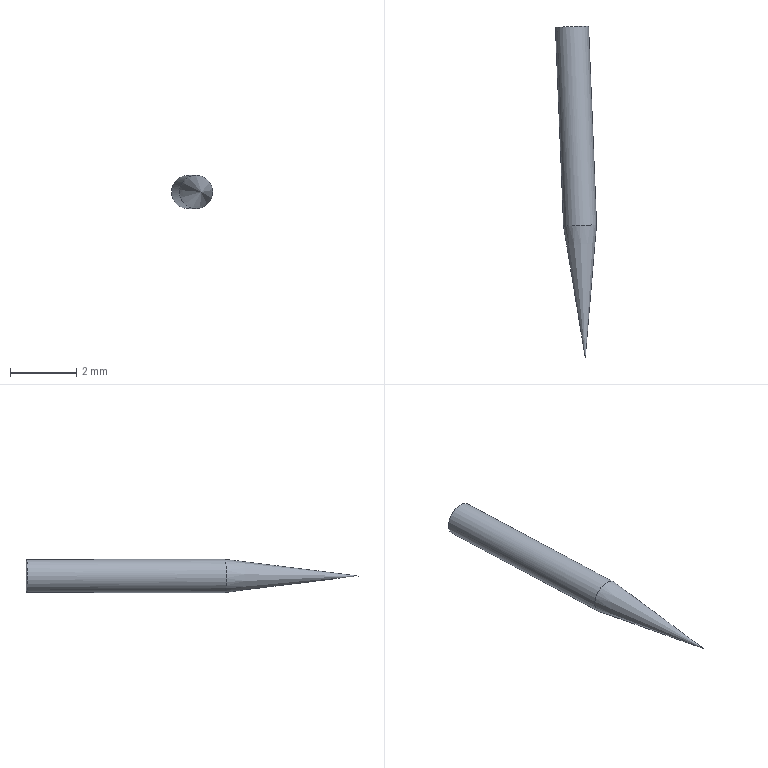Component | NX | 04 | 1 solid | 3 faces | box 1.24 x 10.01 x 1 mm | volume 6 mm3 | plane 1 | cylinder 1 | cone 1 | commonest cylinder face diameters 1 x1
STEP:
#1=CARTESIAN_POINT('',(0.,0.,0.));
#2=DIRECTION('',(0.,0.,1.));
#3=DIRECTION('',(1.,0.,0.));
#4=AXIS2_PLACEMENT_3D('',#1,#2,#3);
#5=CARTESIAN_POINT('',(22.778,-96.137,-0.));
#6=VERTEX_POINT('',#5);
#7=CARTESIAN_POINT('',(22.278,-96.157,-0.));
#8=DIRECTION('',(0.04014,-0.9992,0.));
#9=DIRECTION('',(0.9992,0.04014,0.));
#10=AXIS2_PLACEMENT_3D('',#7,#8,#9);
#11=CIRCLE('',#10,0.5);
#12=CARTESIAN_POINT('',(22.278,-96.157,-0.));
#13=DIRECTION('',(-0.04014,0.9992,0.));
#14=DIRECTION('',(0.,0.,1.));
#15=AXIS2_PLACEMENT_3D('',#12,#13,#14);
#16=PLANE('',#15);
#17=CARTESIAN_POINT('',(0.,0.5));
#18=CARTESIAN_POINT('',(0.866,0.5));
#19=CARTESIAN_POINT('',(0.433,-0.25));
#20=CARTESIAN_POINT('',(0.,-1.));
#21=CARTESIAN_POINT('',(-0.433,-0.25));
#22=CARTESIAN_POINT('',(-0.866,0.5));
#23=CARTESIAN_POINT('',(0.,0.5));
#24=(BOUNDED_CURVE()B_SPLINE_CURVE(2,(#17,#18,#19,#20,#21,#22,#23),.UNSPECIFIED.,.T.,.F.)B_SPLINE_CURVE_WITH_KNOTS((1,2,2,2,2,1),(-2.094,0.,2.094,4.189,6.283,8.378),.UNSPECIFIED.)CURVE()GEOMETRIC_REPRESENTATION_ITEM()RATIONAL_B_SPLINE_CURVE((1.,0.5,1.,0.5,1.,0.5,1.))REPRESENTATION_ITEM(''));
#25=(GEOMETRIC_REPRESENTATION_CONTEXT(2)PARAMETRIC_REPRESENTATION_CONTEXT()REPRESENTATION_CONTEXT('',''));
#26=DEFINITIONAL_REPRESENTATION('',(#24),#25);
#27=PCURVE('',#16,#26);
#28=CARTESIAN_POINT('',(22.278,-96.157,-0.));
#29=DIRECTION('',(0.04014,-0.9992,0.));
#30=DIRECTION('',(0.9992,0.04014,0.));
#31=AXIS2_PLACEMENT_3D('',#28,#29,#30);
#32=CYLINDRICAL_SURFACE('',#31,0.5);
#33=CARTESIAN_POINT('',(0.,0.));
#34=DIRECTION('',(1.,0.));
#35=VECTOR('',#34,1.);
#36=LINE('',#33,#35);
#37=(GEOMETRIC_REPRESENTATION_CONTEXT(2)PARAMETRIC_REPRESENTATION_CONTEXT()REPRESENTATION_CONTEXT('',''));
#38=DEFINITIONAL_REPRESENTATION('',(#36),#37);
#39=PCURVE('',#32,#38);
#40=SURFACE_CURVE('',#11,(#27,#39),.PCURVE_S1.);
#41=EDGE_CURVE('',#6,#6,#40,.T.);
#42=ORIENTED_EDGE('',*,*,#41,.F.);
#43=EDGE_LOOP('',(#42));
#44=FACE_BOUND('',#43,.T.);
#45=ADVANCED_FACE('',(#44),#16,.T.);
#46=CARTESIAN_POINT('',(22.519,-102.153,-0.5));
#47=VERTEX_POINT('',#46);
#48=CARTESIAN_POINT('',(22.519,-102.153,0.5));
#49=VERTEX_POINT('',#48);
#50=CARTESIAN_POINT('',(22.519,-102.153,-0.));
#51=DIRECTION('',(-0.04014,0.9992,0.));
#52=DIRECTION('',(0.,0.,-1.));
#53=AXIS2_PLACEMENT_3D('',#50,#51,#52);
#54=CIRCLE('',#53,0.5);
#55=CARTESIAN_POINT('',(4.712,6.));
#56=DIRECTION('',(-1.,0.));
#57=VECTOR('',#56,1.);
#58=LINE('',#55,#57);
#59=(GEOMETRIC_REPRESENTATION_CONTEXT(2)PARAMETRIC_REPRESENTATION_CONTEXT()REPRESENTATION_CONTEXT('',''));
#60=DEFINITIONAL_REPRESENTATION('',(#58),#59);
#61=PCURVE('',#32,#60);
#62=CARTESIAN_POINT('',(22.519,-102.153,-0.));
#63=DIRECTION('',(-0.04014,0.9992,0.));
#64=DIRECTION('',(0.,0.,1.));
#65=AXIS2_PLACEMENT_3D('',#62,#63,#64);
#66=CONICAL_SURFACE('',#65,0.5,0.1244);
#67=CARTESIAN_POINT('',(3.142,0.));
#68=DIRECTION('',(1.,-0.));
#69=VECTOR('',#68,1.);
#70=LINE('',#67,#69);
#71=(GEOMETRIC_REPRESENTATION_CONTEXT(2)PARAMETRIC_REPRESENTATION_CONTEXT()REPRESENTATION_CONTEXT('',''));
#72=DEFINITIONAL_REPRESENTATION('',(#70),#71);
#73=PCURVE('',#66,#72);
#74=SURFACE_CURVE('',#54,(#61,#73),.PCURVE_S1.);
#75=EDGE_CURVE('',#47,#49,#74,.T.);
#76=ORIENTED_EDGE('',*,*,#75,.T.);
#77=CARTESIAN_POINT('',(23.018,-102.133,-0.));
#78=VERTEX_POINT('',#77);
#79=CARTESIAN_POINT('',(22.519,-102.153,-0.));
#80=DIRECTION('',(-0.04014,0.9992,0.));
#81=DIRECTION('',(0.,0.,-1.));
#82=AXIS2_PLACEMENT_3D('',#79,#80,#81);
#83=CIRCLE('',#82,0.5);
#84=CARTESIAN_POINT('',(4.712,6.));
#85=DIRECTION('',(-1.,0.));
#86=VECTOR('',#85,1.);
#87=LINE('',#84,#86);
#88=(GEOMETRIC_REPRESENTATION_CONTEXT(2)PARAMETRIC_REPRESENTATION_CONTEXT()REPRESENTATION_CONTEXT('',''));
#89=DEFINITIONAL_REPRESENTATION('',(#87),#88);
#90=PCURVE('',#32,#89);
#91=CARTESIAN_POINT('',(-3.142,0.));
#92=DIRECTION('',(1.,-0.));
#93=VECTOR('',#92,1.);
#94=LINE('',#91,#93);
#95=(GEOMETRIC_REPRESENTATION_CONTEXT(2)PARAMETRIC_REPRESENTATION_CONTEXT()REPRESENTATION_CONTEXT('',''));
#96=DEFINITIONAL_REPRESENTATION('',(#94),#95);
#97=PCURVE('',#66,#96);
#98=SURFACE_CURVE('',#83,(#90,#97),.PCURVE_S1.);
#99=EDGE_CURVE('',#49,#78,#98,.T.);
#100=ORIENTED_EDGE('',*,*,#99,.T.);
#101=CARTESIAN_POINT('',(22.778,-96.137,-0.));
#102=CARTESIAN_POINT('',(23.018,-102.133,-0.));
#103=B_SPLINE_CURVE_WITH_KNOTS('',1,(#101,#102),.UNSPECIFIED.,.F.,.F.,(2,2),(0.,6.),.PIECEWISE_BEZIER_KNOTS.);
#104=CARTESIAN_POINT('',(0.,0.));
#105=DIRECTION('',(0.,1.));
#106=VECTOR('',#105,1.);
#107=LINE('',#104,#106);
#108=(GEOMETRIC_REPRESENTATION_CONTEXT(2)PARAMETRIC_REPRESENTATION_CONTEXT()REPRESENTATION_CONTEXT('',''));
#109=DEFINITIONAL_REPRESENTATION('',(#107),#108);
#110=PCURVE('',#32,#109);
#111=CARTESIAN_POINT('',(6.283,0.));
#112=DIRECTION('',(0.,1.));
#113=VECTOR('',#112,1.);
#114=LINE('',#111,#113);
#115=(GEOMETRIC_REPRESENTATION_CONTEXT(2)PARAMETRIC_REPRESENTATION_CONTEXT()REPRESENTATION_CONTEXT('',''));
#116=DEFINITIONAL_REPRESENTATION('',(#114),#115);
#117=PCURVE('',#32,#116);
#118=SEAM_CURVE('',#103,(#110,#117),.PCURVE_S1.);
#119=EDGE_CURVE('',#6,#78,#118,.T.);
#120=ORIENTED_EDGE('',*,*,#119,.F.);
#121=ORIENTED_EDGE('',*,*,#41,.T.);
#122=ORIENTED_EDGE('',*,*,#119,.T.);
#123=CARTESIAN_POINT('',(22.519,-102.153,-0.));
#124=DIRECTION('',(-0.04014,0.9992,0.));
#125=DIRECTION('',(0.,0.,-1.));
#126=AXIS2_PLACEMENT_3D('',#123,#124,#125);
#127=CIRCLE('',#126,0.5);
#128=CARTESIAN_POINT('',(10.996,6.));
#129=DIRECTION('',(-1.,0.));
#130=VECTOR('',#129,1.);
#131=LINE('',#128,#130);
#132=(GEOMETRIC_REPRESENTATION_CONTEXT(2)PARAMETRIC_REPRESENTATION_CONTEXT()REPRESENTATION_CONTEXT('',''));
#133=DEFINITIONAL_REPRESENTATION('',(#131),#132);
#134=PCURVE('',#32,#133);
#135=CARTESIAN_POINT('',(-3.142,-0.));
#136=DIRECTION('',(1.,0.));
#137=VECTOR('',#136,1.);
#138=LINE('',#135,#137);
#139=(GEOMETRIC_REPRESENTATION_CONTEXT(2)PARAMETRIC_REPRESENTATION_CONTEXT()REPRESENTATION_CONTEXT('',''));
#140=DEFINITIONAL_REPRESENTATION('',(#138),#139);
#141=PCURVE('',#66,#140);
#142=SURFACE_CURVE('',#127,(#134,#141),.PCURVE_S1.);
#143=EDGE_CURVE('',#78,#47,#142,.T.);
#144=ORIENTED_EDGE('',*,*,#143,.T.);
#145=EDGE_LOOP('',(#76,#100,#120,#121,#122,#144));
#146=FACE_BOUND('',#145,.T.);
#147=ADVANCED_FACE('',(#146),#32,.T.);
#148=CARTESIAN_POINT('',(22.679,-106.149,-0.));
#149=VERTEX_POINT('',#148);
#150=CARTESIAN_POINT('',(22.679,-106.149,-0.));
#151=CARTESIAN_POINT('',(22.519,-102.153,0.5));
#152=B_SPLINE_CURVE_WITH_KNOTS('',1,(#150,#151),.UNSPECIFIED.,.F.,.F.,(2,2),(-4.031,-0.),.PIECEWISE_BEZIER_KNOTS.);
#153=CARTESIAN_POINT('',(6.283,0.));
#154=DIRECTION('',(0.,1.));
#155=VECTOR('',#154,1.);
#156=LINE('',#153,#155);
#157=(GEOMETRIC_REPRESENTATION_CONTEXT(2)PARAMETRIC_REPRESENTATION_CONTEXT()REPRESENTATION_CONTEXT('',''));
#158=DEFINITIONAL_REPRESENTATION('',(#156),#157);
#159=PCURVE('',#66,#158);
#160=CARTESIAN_POINT('',(0.,0.));
#161=DIRECTION('',(0.,1.));
#162=VECTOR('',#161,1.);
#163=LINE('',#160,#162);
#164=(GEOMETRIC_REPRESENTATION_CONTEXT(2)PARAMETRIC_REPRESENTATION_CONTEXT()REPRESENTATION_CONTEXT('',''));
#165=DEFINITIONAL_REPRESENTATION('',(#163),#164);
#166=PCURVE('',#66,#165);
#167=SEAM_CURVE('',#152,(#159,#166),.PCURVE_S1.);
#168=EDGE_CURVE('',#149,#49,#167,.T.);
#169=ORIENTED_EDGE('',*,*,#168,.T.);
#170=ORIENTED_EDGE('',*,*,#75,.F.);
#171=ORIENTED_EDGE('',*,*,#143,.F.);
#172=ORIENTED_EDGE('',*,*,#99,.F.);
#173=ORIENTED_EDGE('',*,*,#168,.F.);
#174=EDGE_LOOP('',(#169,#170,#171,#172,#173));
#175=FACE_BOUND('',#174,.T.);
#176=ADVANCED_FACE('',(#175),#66,.T.);
#177=CLOSED_SHELL('',(#45,#147,#176));
#178=MANIFOLD_SOLID_BREP('',#177);
#179=(LENGTH_UNIT()NAMED_UNIT(*)SI_UNIT(.MILLI.,.METRE.));
#180=UNCERTAINTY_MEASURE_WITH_UNIT(LENGTH_MEASURE(0.000005),#179,'','');
#181=(NAMED_UNIT(*)PLANE_ANGLE_UNIT()SI_UNIT($,.RADIAN.));
#182=(NAMED_UNIT(*)SI_UNIT($,.STERADIAN.)SOLID_ANGLE_UNIT());
#183=(GEOMETRIC_REPRESENTATION_CONTEXT(3)GLOBAL_UNCERTAINTY_ASSIGNED_CONTEXT((#180))GLOBAL_UNIT_ASSIGNED_CONTEXT((#179,#181,#182))REPRESENTATION_CONTEXT('',''));
#184=ADVANCED_BREP_SHAPE_REPRESENTATION('',(#4,#178),#183);